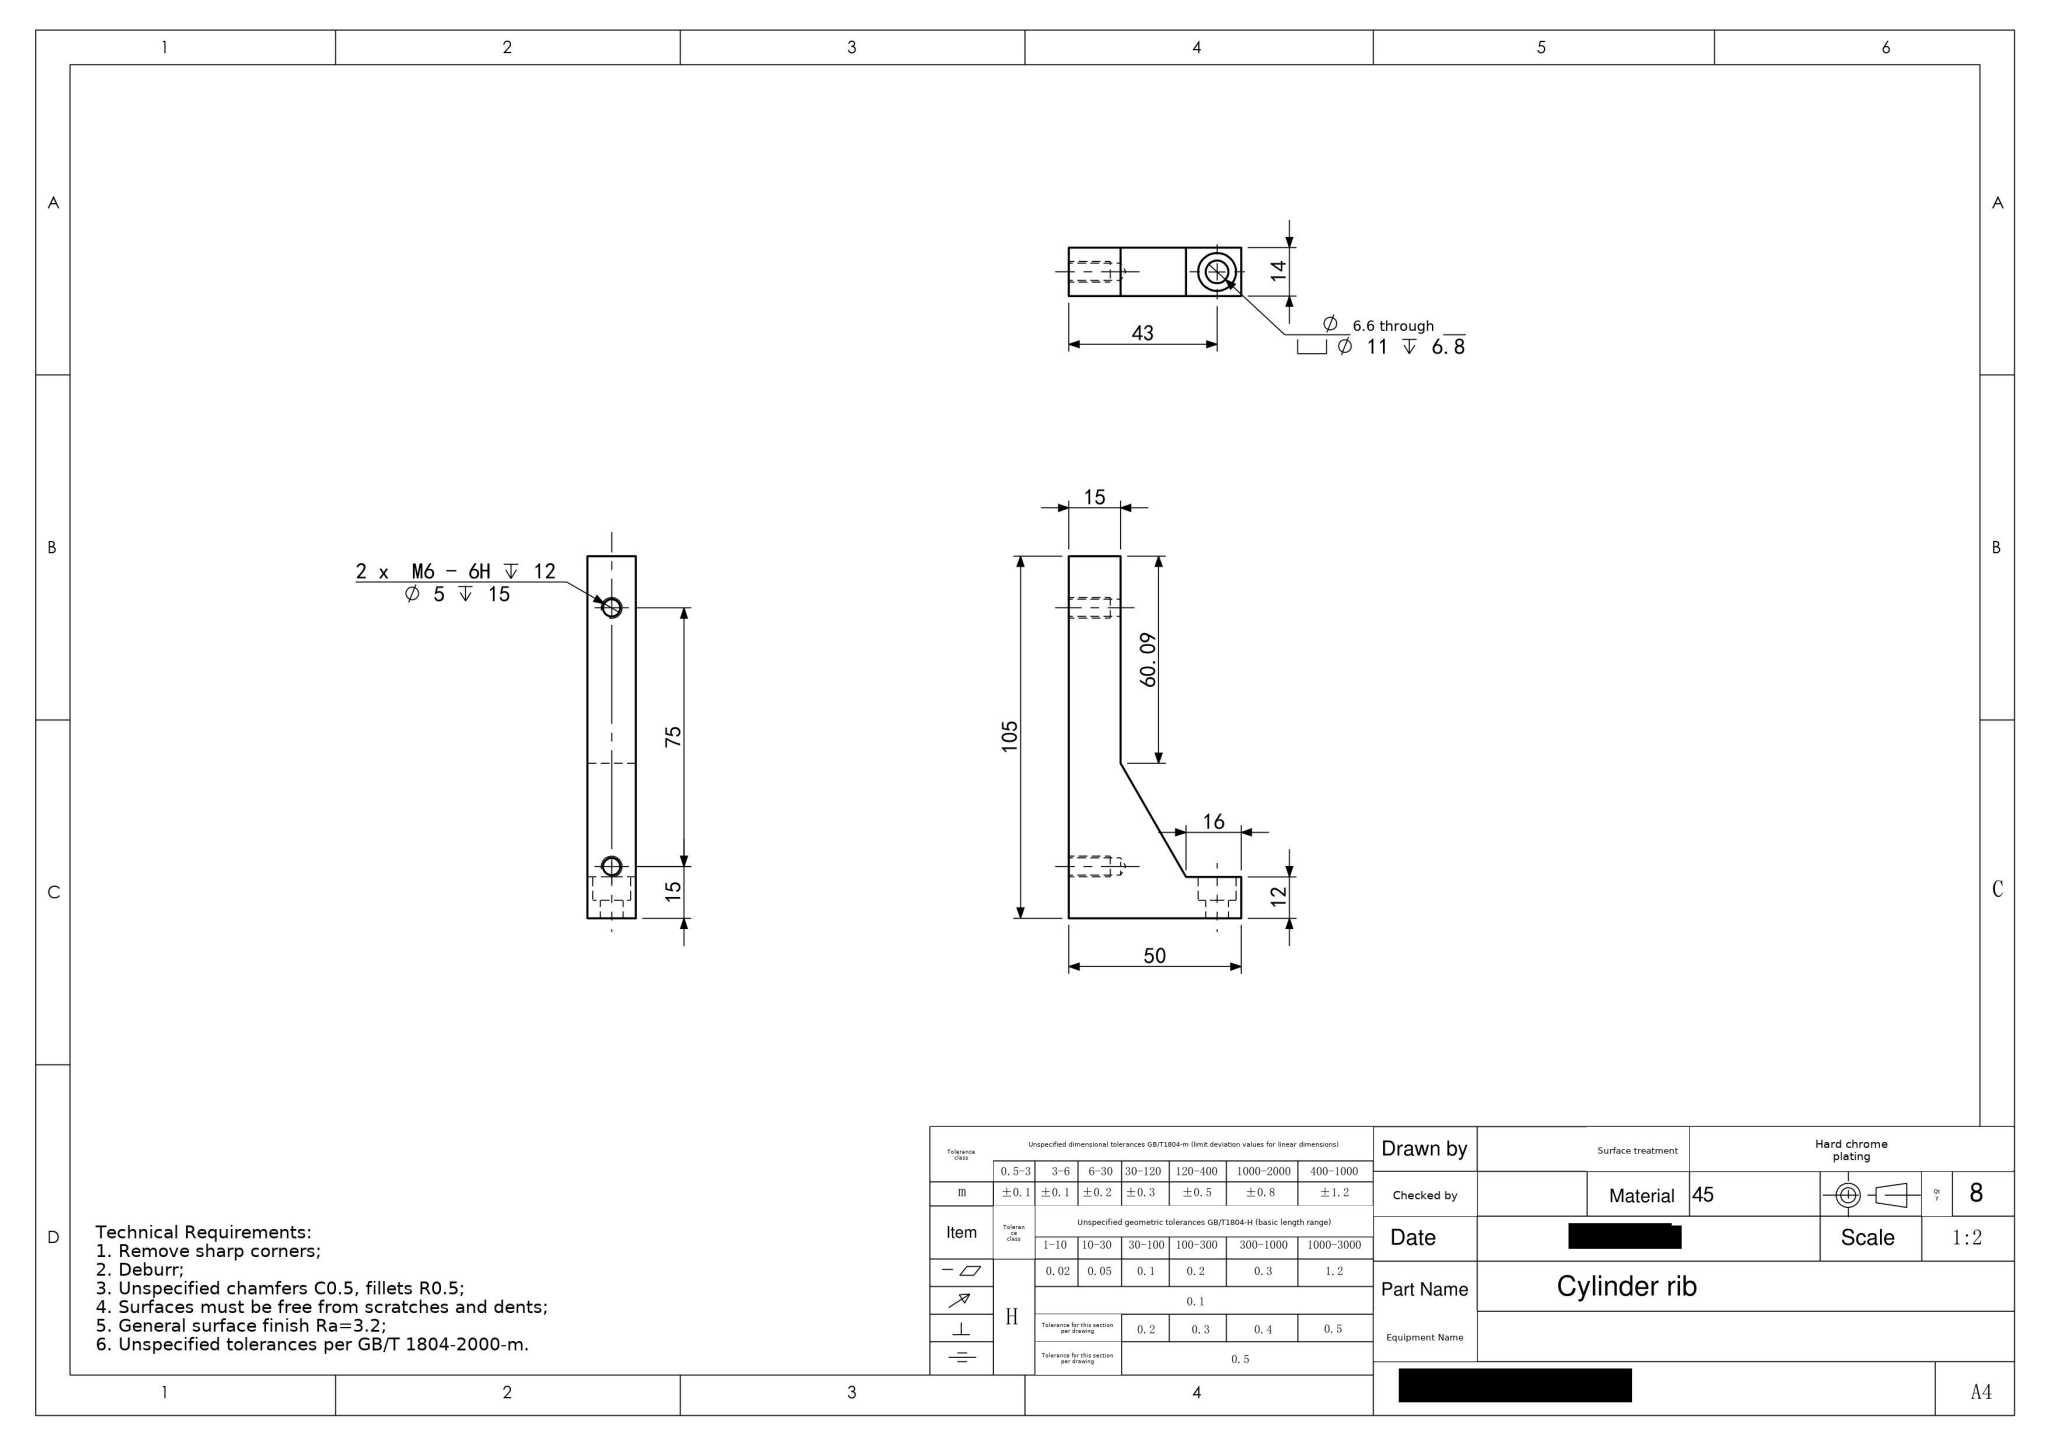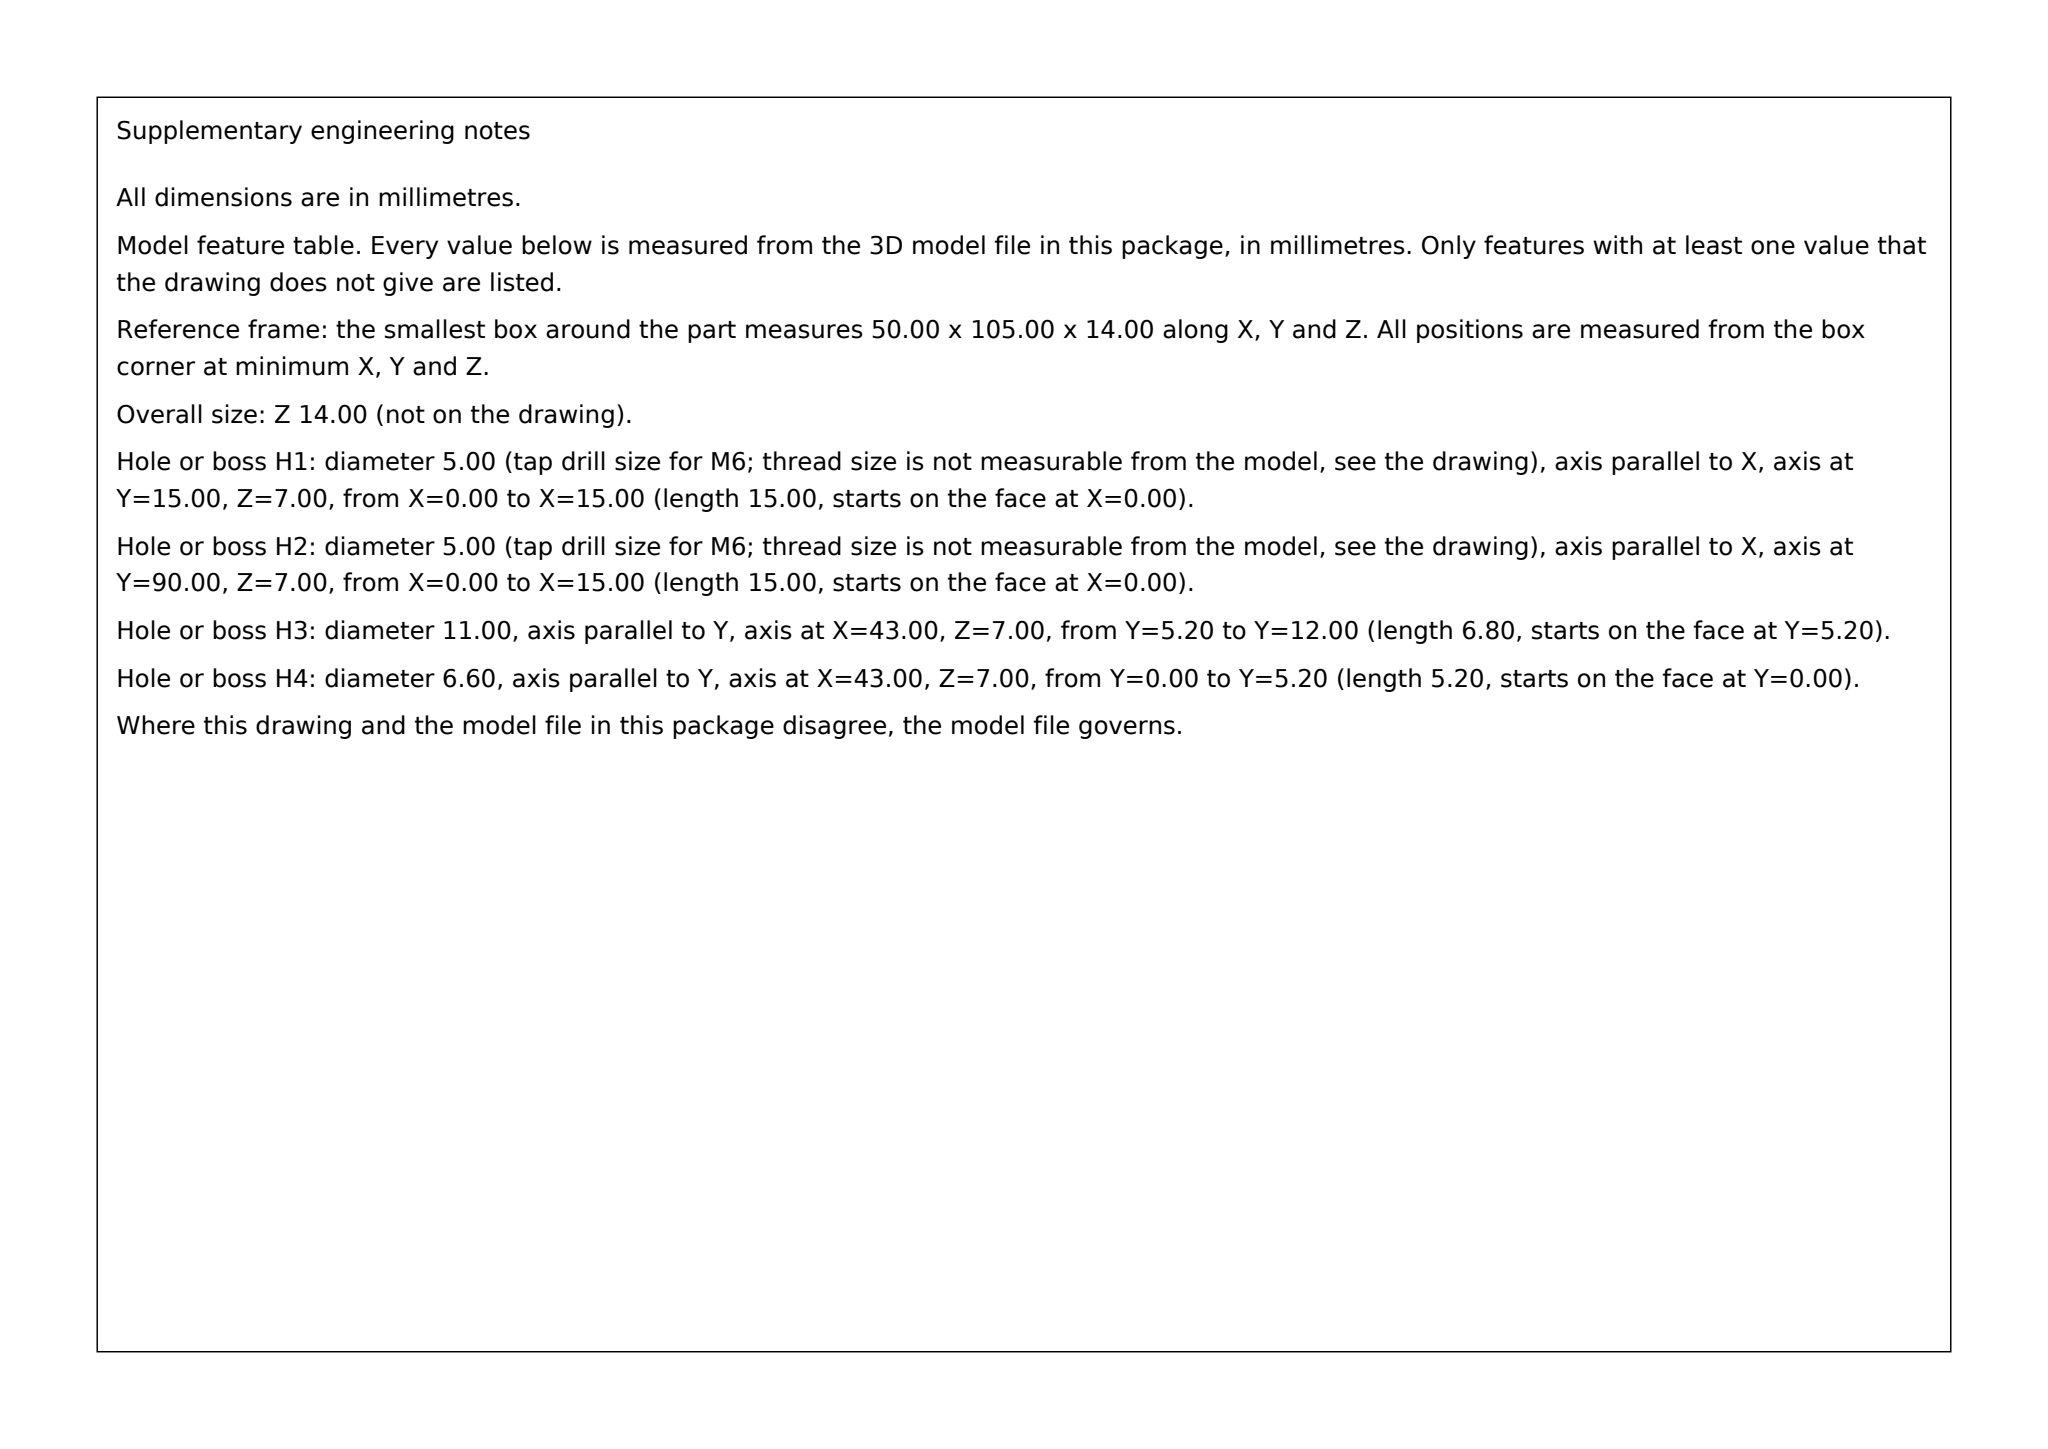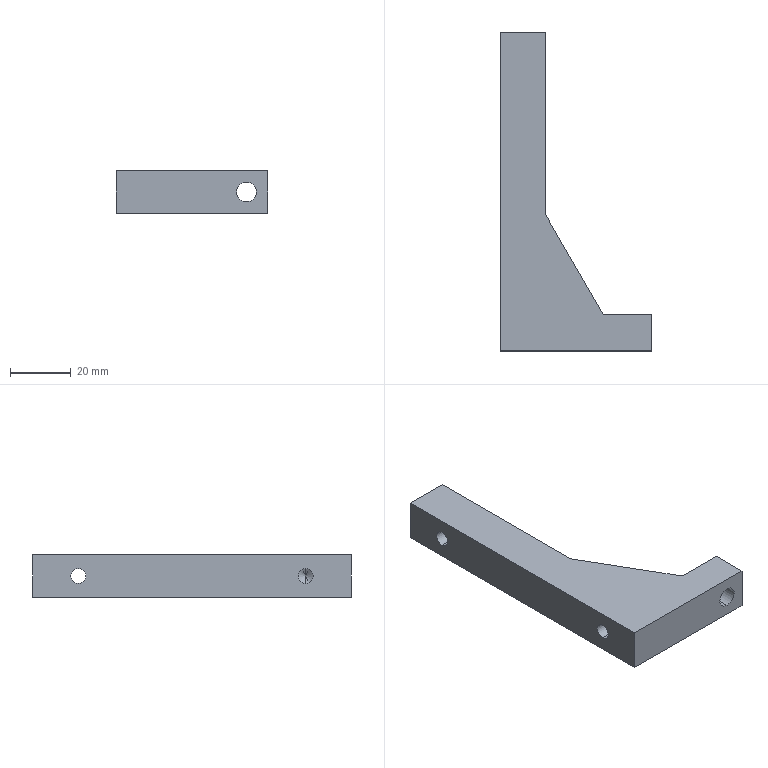Part | SolidWorks | mm | material 45 | 1 solid | 20 faces | box 50 x 105 x 14 mm | volume 30884 mm3 | plane 10 | cylinder 8 | cone 2 | commonest cylinder face diameters 5 x4 11 x2 6.6 x2
build123d program:
from build123d import *

# Parameters (mm, degrees)
BOSS_EXTRUDE1_DEPTH                             = 7
M6_HEX_SOCKET_HEAD_CAP_SCREW_CBORE1_D           = 6.6
M6_HEX_SOCKET_HEAD_CAP_SCREW_CBORE1_CBORE_D     = 11
M6_HEX_SOCKET_HEAD_CAP_SCREW_CBORE1_CBORE_DEPTH = 6.8
LPATTERN1_COUNT                                 = 2
LPATTERN1_PITCH                                 = 75


with BuildPart() as part:
    # Sketch1 → Boss-Extrude1 (new, symmetric)
    with BuildSketch(Plane.XY):
        Polygon((-25, 0), (25, 0), (25, 12), (9, 12), (-10, 44.909), (-10, 105), (-25, 105), align=None)
    extrude(amount=BOSS_EXTRUDE1_DEPTH, both=True)

    # M6 Hex Socket Head Cap Screw CBORE1 (through all)
    with Locations(Plane(origin=(0, 12, 0), x_dir=(1, 0, 0), z_dir=(0, 1, 0))):
        with Locations((18, 0)):
            CounterBoreHole(M6_HEX_SOCKET_HEAD_CAP_SCREW_CBORE1_D / 2, M6_HEX_SOCKET_HEAD_CAP_SCREW_CBORE1_CBORE_D / 2, M6_HEX_SOCKET_HEAD_CAP_SCREW_CBORE1_CBORE_DEPTH)

    # Sketch5 → M6 Tapped Hole1 (revolve, cut)
    with BuildSketch(Plane(origin=(-25, 90, 0), x_dir=(0, 0, 1), z_dir=(0, 1, 0))):
        Polygon((0, 0), (0, 16.502), (2.5, 15), (2.5, 0), align=None)
    m6_tapped_hole1 = revolve(axis=Axis((-31.35, 90, 0), (1, 0, 0)), mode=Mode.SUBTRACT)

    # LPattern1: M6 Tapped Hole1 ×2
    with Locations(*[(0, -i * LPATTERN1_PITCH, 0) for i in range(1, LPATTERN1_COUNT)]):
        add(m6_tapped_hole1, mode=Mode.SUBTRACT)


solid = part.part
STEP:
#1=CARTESIAN_POINT('',(-10.,15.,-2.5));
#2=VERTEX_POINT('',#1);
#3=CARTESIAN_POINT('',(-10.,15.,2.5));
#4=VERTEX_POINT('',#3);
#5=CARTESIAN_POINT('',(-10.,15.,0.));
#6=DIRECTION('',(-1.,0.,0.));
#7=DIRECTION('',(0.,0.,1.));
#8=AXIS2_PLACEMENT_3D('',#5,#6,#7);
#9=CIRCLE('',#8,2.5);
#10=EDGE_CURVE('',#2,#4,#9,.T.);
#11=ORIENTED_EDGE('',*,*,#10,.F.);
#12=CARTESIAN_POINT('',(-25.,15.,-2.5));
#13=VERTEX_POINT('',#12);
#14=CARTESIAN_POINT('',(-25.,15.,-2.5));
#15=DIRECTION('',(-1.,0.,0.));
#16=VECTOR('',#15,1000.);
#17=LINE('',#14,#16);
#18=EDGE_CURVE('',#2,#13,#17,.T.);
#19=ORIENTED_EDGE('',*,*,#18,.T.);
#20=CARTESIAN_POINT('',(-25.,15.,2.5));
#21=VERTEX_POINT('',#20);
#22=CARTESIAN_POINT('',(-25.,15.,0.));
#23=DIRECTION('',(-1.,0.,0.));
#24=DIRECTION('',(0.,0.,1.));
#25=AXIS2_PLACEMENT_3D('',#22,#23,#24);
#26=CIRCLE('',#25,2.5);
#27=EDGE_CURVE('',#13,#21,#26,.T.);
#28=ORIENTED_EDGE('',*,*,#27,.T.);
#29=CARTESIAN_POINT('',(-25.,15.,2.5));
#30=DIRECTION('',(-1.,0.,0.));
#31=VECTOR('',#30,1000.);
#32=LINE('',#29,#31);
#33=EDGE_CURVE('',#4,#21,#32,.T.);
#34=ORIENTED_EDGE('',*,*,#33,.F.);
#35=EDGE_LOOP('',(#11,#19,#28,#34));
#36=FACE_OUTER_BOUND('',#35,.T.);
#37=CARTESIAN_POINT('',(-25.,15.,0.));
#38=DIRECTION('',(-1.,0.,0.));
#39=DIRECTION('',(0.,0.,1.));
#40=AXIS2_PLACEMENT_3D('',#37,#38,#39);
#41=CYLINDRICAL_SURFACE('',#40,2.5);
#42=ADVANCED_FACE('',(#36),#41,.F.);
#43=CARTESIAN_POINT('',(-8.498,15.,0.));
#44=VERTEX_POINT('',#43);
#45=CARTESIAN_POINT('',(-10.,15.,2.5));
#46=DIRECTION('',(-0.515,0.,0.8572));
#47=VECTOR('',#46,1000.);
#48=LINE('',#45,#47);
#49=EDGE_CURVE('',#44,#4,#48,.T.);
#50=ORIENTED_EDGE('',*,*,#49,.F.);
#51=CARTESIAN_POINT('',(-10.,15.,-2.5));
#52=DIRECTION('',(-0.515,0.,-0.8572));
#53=VECTOR('',#52,1000.);
#54=LINE('',#51,#53);
#55=EDGE_CURVE('',#44,#2,#54,.T.);
#56=ORIENTED_EDGE('',*,*,#55,.T.);
#57=ORIENTED_EDGE('',*,*,#10,.T.);
#58=EDGE_LOOP('',(#50,#56,#57));
#59=FACE_OUTER_BOUND('',#58,.T.);
#60=CARTESIAN_POINT('',(-10.,15.,0.));
#61=DIRECTION('',(-1.,0.,0.));
#62=DIRECTION('',(0.,0.,1.));
#63=AXIS2_PLACEMENT_3D('',#60,#61,#62);
#64=CONICAL_SURFACE('',#63,2.5,1.03);
#65=ADVANCED_FACE('',(#59),#64,.F.);
#66=CARTESIAN_POINT('',(-10.,90.,-2.5));
#67=VERTEX_POINT('',#66);
#68=CARTESIAN_POINT('',(-10.,90.,2.5));
#69=VERTEX_POINT('',#68);
#70=CARTESIAN_POINT('',(-10.,90.,0.));
#71=DIRECTION('',(-1.,0.,0.));
#72=DIRECTION('',(0.,0.,1.));
#73=AXIS2_PLACEMENT_3D('',#70,#71,#72);
#74=CIRCLE('',#73,2.5);
#75=EDGE_CURVE('',#67,#69,#74,.T.);
#76=ORIENTED_EDGE('',*,*,#75,.F.);
#77=CARTESIAN_POINT('',(-25.,90.,-2.5));
#78=VERTEX_POINT('',#77);
#79=CARTESIAN_POINT('',(-25.,90.,-2.5));
#80=DIRECTION('',(-1.,0.,0.));
#81=VECTOR('',#80,1000.);
#82=LINE('',#79,#81);
#83=EDGE_CURVE('',#67,#78,#82,.T.);
#84=ORIENTED_EDGE('',*,*,#83,.T.);
#85=CARTESIAN_POINT('',(-25.,90.,2.5));
#86=VERTEX_POINT('',#85);
#87=CARTESIAN_POINT('',(-25.,90.,0.));
#88=DIRECTION('',(-1.,0.,0.));
#89=DIRECTION('',(0.,0.,1.));
#90=AXIS2_PLACEMENT_3D('',#87,#88,#89);
#91=CIRCLE('',#90,2.5);
#92=EDGE_CURVE('',#78,#86,#91,.T.);
#93=ORIENTED_EDGE('',*,*,#92,.T.);
#94=CARTESIAN_POINT('',(-25.,90.,2.5));
#95=DIRECTION('',(-1.,0.,0.));
#96=VECTOR('',#95,1000.);
#97=LINE('',#94,#96);
#98=EDGE_CURVE('',#69,#86,#97,.T.);
#99=ORIENTED_EDGE('',*,*,#98,.F.);
#100=EDGE_LOOP('',(#76,#84,#93,#99));
#101=FACE_OUTER_BOUND('',#100,.T.);
#102=CARTESIAN_POINT('',(-25.,90.,0.));
#103=DIRECTION('',(-1.,0.,0.));
#104=DIRECTION('',(0.,0.,1.));
#105=AXIS2_PLACEMENT_3D('',#102,#103,#104);
#106=CYLINDRICAL_SURFACE('',#105,2.5);
#107=ADVANCED_FACE('',(#101),#106,.F.);
#108=CARTESIAN_POINT('',(18.,5.2,-5.5));
#109=VERTEX_POINT('',#108);
#110=CARTESIAN_POINT('',(18.,5.2,5.5));
#111=VERTEX_POINT('',#110);
#112=CARTESIAN_POINT('',(18.,5.2,0.));
#113=DIRECTION('',(0.,1.,0.));
#114=DIRECTION('',(0.,0.,1.));
#115=AXIS2_PLACEMENT_3D('',#112,#113,#114);
#116=CIRCLE('',#115,5.5);
#117=EDGE_CURVE('',#109,#111,#116,.T.);
#118=ORIENTED_EDGE('',*,*,#117,.F.);
#119=CARTESIAN_POINT('',(18.,12.,-5.5));
#120=VERTEX_POINT('',#119);
#121=CARTESIAN_POINT('',(18.,12.,-5.5));
#122=DIRECTION('',(0.,1.,0.));
#123=VECTOR('',#122,1000.);
#124=LINE('',#121,#123);
#125=EDGE_CURVE('',#109,#120,#124,.T.);
#126=ORIENTED_EDGE('',*,*,#125,.T.);
#127=CARTESIAN_POINT('',(18.,12.,5.5));
#128=VERTEX_POINT('',#127);
#129=CARTESIAN_POINT('',(18.,12.,0.));
#130=DIRECTION('',(0.,1.,0.));
#131=DIRECTION('',(0.,0.,1.));
#132=AXIS2_PLACEMENT_3D('',#129,#130,#131);
#133=CIRCLE('',#132,5.5);
#134=EDGE_CURVE('',#120,#128,#133,.T.);
#135=ORIENTED_EDGE('',*,*,#134,.T.);
#136=CARTESIAN_POINT('',(18.,12.,5.5));
#137=DIRECTION('',(0.,1.,0.));
#138=VECTOR('',#137,1000.);
#139=LINE('',#136,#138);
#140=EDGE_CURVE('',#111,#128,#139,.T.);
#141=ORIENTED_EDGE('',*,*,#140,.F.);
#142=EDGE_LOOP('',(#118,#126,#135,#141));
#143=FACE_OUTER_BOUND('',#142,.T.);
#144=CARTESIAN_POINT('',(18.,12.,0.));
#145=DIRECTION('',(0.,1.,0.));
#146=DIRECTION('',(0.,0.,1.));
#147=AXIS2_PLACEMENT_3D('',#144,#145,#146);
#148=CYLINDRICAL_SURFACE('',#147,5.5);
#149=ADVANCED_FACE('',(#143),#148,.F.);
#150=CARTESIAN_POINT('',(18.,0.,-3.3));
#151=VERTEX_POINT('',#150);
#152=CARTESIAN_POINT('',(18.,0.,3.3));
#153=VERTEX_POINT('',#152);
#154=CARTESIAN_POINT('',(18.,0.,0.));
#155=DIRECTION('',(-0.,1.,0.));
#156=DIRECTION('',(-1.,-0.,0.));
#157=AXIS2_PLACEMENT_3D('',#154,#155,#156);
#158=CIRCLE('',#157,3.3);
#159=EDGE_CURVE('',#151,#153,#158,.T.);
#160=ORIENTED_EDGE('',*,*,#159,.F.);
#161=CARTESIAN_POINT('',(18.,5.2,-3.3));
#162=VERTEX_POINT('',#161);
#163=CARTESIAN_POINT('',(18.,12.,-3.3));
#164=DIRECTION('',(0.,1.,0.));
#165=VECTOR('',#164,1000.);
#166=LINE('',#163,#165);
#167=EDGE_CURVE('',#151,#162,#166,.T.);
#168=ORIENTED_EDGE('',*,*,#167,.T.);
#169=CARTESIAN_POINT('',(18.,5.2,3.3));
#170=VERTEX_POINT('',#169);
#171=CARTESIAN_POINT('',(18.,5.2,0.));
#172=DIRECTION('',(0.,1.,0.));
#173=DIRECTION('',(0.,0.,1.));
#174=AXIS2_PLACEMENT_3D('',#171,#172,#173);
#175=CIRCLE('',#174,3.3);
#176=EDGE_CURVE('',#162,#170,#175,.T.);
#177=ORIENTED_EDGE('',*,*,#176,.T.);
#178=CARTESIAN_POINT('',(18.,12.,3.3));
#179=DIRECTION('',(0.,1.,0.));
#180=VECTOR('',#179,1000.);
#181=LINE('',#178,#180);
#182=EDGE_CURVE('',#153,#170,#181,.T.);
#183=ORIENTED_EDGE('',*,*,#182,.F.);
#184=EDGE_LOOP('',(#160,#168,#177,#183));
#185=FACE_OUTER_BOUND('',#184,.T.);
#186=CARTESIAN_POINT('',(18.,12.,0.));
#187=DIRECTION('',(0.,1.,0.));
#188=DIRECTION('',(0.,0.,1.));
#189=AXIS2_PLACEMENT_3D('',#186,#187,#188);
#190=CYLINDRICAL_SURFACE('',#189,3.3);
#191=ADVANCED_FACE('',(#185),#190,.F.);
#192=CARTESIAN_POINT('',(-25.,15.,0.));
#193=DIRECTION('',(-1.,0.,0.));
#194=DIRECTION('',(0.,0.,1.));
#195=AXIS2_PLACEMENT_3D('',#192,#193,#194);
#196=CIRCLE('',#195,2.5);
#197=EDGE_CURVE('',#21,#13,#196,.T.);
#198=ORIENTED_EDGE('',*,*,#197,.F.);
#199=ORIENTED_EDGE('',*,*,#27,.F.);
#200=EDGE_LOOP('',(#198,#199));
#201=FACE_BOUND('',#200,.T.);
#202=CARTESIAN_POINT('',(-25.,90.,0.));
#203=DIRECTION('',(-1.,0.,0.));
#204=DIRECTION('',(0.,0.,1.));
#205=AXIS2_PLACEMENT_3D('',#202,#203,#204);
#206=CIRCLE('',#205,2.5);
#207=EDGE_CURVE('',#86,#78,#206,.T.);
#208=ORIENTED_EDGE('',*,*,#207,.F.);
#209=ORIENTED_EDGE('',*,*,#92,.F.);
#210=EDGE_LOOP('',(#208,#209));
#211=FACE_BOUND('',#210,.T.);
#212=CARTESIAN_POINT('',(-25.,105.,-7.));
#213=VERTEX_POINT('',#212);
#214=CARTESIAN_POINT('',(-25.,0.,-7.));
#215=VERTEX_POINT('',#214);
#216=CARTESIAN_POINT('',(-25.,0.,-7.));
#217=DIRECTION('',(0.,-1.,0.));
#218=VECTOR('',#217,1000.);
#219=LINE('',#216,#218);
#220=EDGE_CURVE('',#213,#215,#219,.T.);
#221=ORIENTED_EDGE('',*,*,#220,.T.);
#222=CARTESIAN_POINT('',(-25.,0.,7.));
#223=VERTEX_POINT('',#222);
#224=CARTESIAN_POINT('',(-25.,0.,7.));
#225=DIRECTION('',(0.,0.,-1.));
#226=VECTOR('',#225,1000.);
#227=LINE('',#224,#226);
#228=EDGE_CURVE('',#223,#215,#227,.T.);
#229=ORIENTED_EDGE('',*,*,#228,.F.);
#230=CARTESIAN_POINT('',(-25.,105.,7.));
#231=VERTEX_POINT('',#230);
#232=CARTESIAN_POINT('',(-25.,0.,7.));
#233=DIRECTION('',(0.,-1.,0.));
#234=VECTOR('',#233,1000.);
#235=LINE('',#232,#234);
#236=EDGE_CURVE('',#231,#223,#235,.T.);
#237=ORIENTED_EDGE('',*,*,#236,.F.);
#238=CARTESIAN_POINT('',(-25.,105.,7.));
#239=DIRECTION('',(0.,0.,-1.));
#240=VECTOR('',#239,1000.);
#241=LINE('',#238,#240);
#242=EDGE_CURVE('',#231,#213,#241,.T.);
#243=ORIENTED_EDGE('',*,*,#242,.T.);
#244=EDGE_LOOP('',(#221,#229,#237,#243));
#245=FACE_OUTER_BOUND('',#244,.T.);
#246=CARTESIAN_POINT('',(-25.,0.,7.));
#247=DIRECTION('',(1.,0.,0.));
#248=DIRECTION('',(0.,0.,-1.));
#249=AXIS2_PLACEMENT_3D('',#246,#247,#248);
#250=PLANE('',#249);
#251=ADVANCED_FACE('',(#201,#211,#245),#250,.F.);
#252=CARTESIAN_POINT('',(18.,0.,0.));
#253=DIRECTION('',(-0.,1.,0.));
#254=DIRECTION('',(-1.,-0.,0.));
#255=AXIS2_PLACEMENT_3D('',#252,#253,#254);
#256=CIRCLE('',#255,3.3);
#257=EDGE_CURVE('',#153,#151,#256,.T.);
#258=ORIENTED_EDGE('',*,*,#257,.T.);
#259=ORIENTED_EDGE('',*,*,#159,.T.);
#260=EDGE_LOOP('',(#258,#259));
#261=FACE_BOUND('',#260,.T.);
#262=CARTESIAN_POINT('',(25.,0.,-7.));
#263=VERTEX_POINT('',#262);
#264=CARTESIAN_POINT('',(-25.,0.,-7.));
#265=DIRECTION('',(1.,0.,0.));
#266=VECTOR('',#265,1000.);
#267=LINE('',#264,#266);
#268=EDGE_CURVE('',#215,#263,#267,.T.);
#269=ORIENTED_EDGE('',*,*,#268,.T.);
#270=CARTESIAN_POINT('',(25.,0.,7.));
#271=VERTEX_POINT('',#270);
#272=CARTESIAN_POINT('',(25.,0.,7.));
#273=DIRECTION('',(0.,0.,-1.));
#274=VECTOR('',#273,1000.);
#275=LINE('',#272,#274);
#276=EDGE_CURVE('',#271,#263,#275,.T.);
#277=ORIENTED_EDGE('',*,*,#276,.F.);
#278=CARTESIAN_POINT('',(-25.,0.,7.));
#279=DIRECTION('',(1.,0.,0.));
#280=VECTOR('',#279,1000.);
#281=LINE('',#278,#280);
#282=EDGE_CURVE('',#223,#271,#281,.T.);
#283=ORIENTED_EDGE('',*,*,#282,.F.);
#284=ORIENTED_EDGE('',*,*,#228,.T.);
#285=EDGE_LOOP('',(#269,#277,#283,#284));
#286=FACE_OUTER_BOUND('',#285,.T.);
#287=CARTESIAN_POINT('',(-25.,0.,7.));
#288=DIRECTION('',(-0.,1.,0.));
#289=DIRECTION('',(-1.,-0.,0.));
#290=AXIS2_PLACEMENT_3D('',#287,#288,#289);
#291=PLANE('',#290);
#292=ADVANCED_FACE('',(#261,#286),#291,.F.);
#293=CARTESIAN_POINT('',(25.,12.,-7.));
#294=VERTEX_POINT('',#293);
#295=CARTESIAN_POINT('',(25.,0.,-7.));
#296=DIRECTION('',(0.,1.,0.));
#297=VECTOR('',#296,1000.);
#298=LINE('',#295,#297);
#299=EDGE_CURVE('',#263,#294,#298,.T.);
#300=ORIENTED_EDGE('',*,*,#299,.T.);
#301=CARTESIAN_POINT('',(25.,12.,7.));
#302=VERTEX_POINT('',#301);
#303=CARTESIAN_POINT('',(25.,12.,7.));
#304=DIRECTION('',(0.,0.,-1.));
#305=VECTOR('',#304,1000.);
#306=LINE('',#303,#305);
#307=EDGE_CURVE('',#302,#294,#306,.T.);
#308=ORIENTED_EDGE('',*,*,#307,.F.);
#309=CARTESIAN_POINT('',(25.,0.,7.));
#310=DIRECTION('',(0.,1.,0.));
#311=VECTOR('',#310,1000.);
#312=LINE('',#309,#311);
#313=EDGE_CURVE('',#271,#302,#312,.T.);
#314=ORIENTED_EDGE('',*,*,#313,.F.);
#315=ORIENTED_EDGE('',*,*,#276,.T.);
#316=EDGE_LOOP('',(#300,#308,#314,#315));
#317=FACE_OUTER_BOUND('',#316,.T.);
#318=CARTESIAN_POINT('',(25.,0.,7.));
#319=DIRECTION('',(-1.,0.,0.));
#320=DIRECTION('',(-0.,-1.,0.));
#321=AXIS2_PLACEMENT_3D('',#318,#319,#320);
#322=PLANE('',#321);
#323=ADVANCED_FACE('',(#317),#322,.F.);
#324=CARTESIAN_POINT('',(18.,12.,0.));
#325=DIRECTION('',(0.,1.,0.));
#326=DIRECTION('',(0.,0.,1.));
#327=AXIS2_PLACEMENT_3D('',#324,#325,#326);
#328=CIRCLE('',#327,5.5);
#329=EDGE_CURVE('',#128,#120,#328,.T.);
#330=ORIENTED_EDGE('',*,*,#329,.F.);
#331=ORIENTED_EDGE('',*,*,#134,.F.);
#332=EDGE_LOOP('',(#330,#331));
#333=FACE_BOUND('',#332,.T.);
#334=CARTESIAN_POINT('',(9.,12.,-7.));
#335=VERTEX_POINT('',#334);
#336=CARTESIAN_POINT('',(9.,12.,-7.));
#337=DIRECTION('',(-1.,0.,0.));
#338=VECTOR('',#337,1000.);
#339=LINE('',#336,#338);
#340=EDGE_CURVE('',#294,#335,#339,.T.);
#341=ORIENTED_EDGE('',*,*,#340,.T.);
#342=CARTESIAN_POINT('',(9.,12.,7.));
#343=VERTEX_POINT('',#342);
#344=CARTESIAN_POINT('',(9.,12.,7.));
#345=DIRECTION('',(0.,0.,-1.));
#346=VECTOR('',#345,1000.);
#347=LINE('',#344,#346);
#348=EDGE_CURVE('',#343,#335,#347,.T.);
#349=ORIENTED_EDGE('',*,*,#348,.F.);
#350=CARTESIAN_POINT('',(9.,12.,7.));
#351=DIRECTION('',(-1.,0.,0.));
#352=VECTOR('',#351,1000.);
#353=LINE('',#350,#352);
#354=EDGE_CURVE('',#302,#343,#353,.T.);
#355=ORIENTED_EDGE('',*,*,#354,.F.);
#356=ORIENTED_EDGE('',*,*,#307,.T.);
#357=EDGE_LOOP('',(#341,#349,#355,#356));
#358=FACE_OUTER_BOUND('',#357,.T.);
#359=CARTESIAN_POINT('',(9.,12.,7.));
#360=DIRECTION('',(0.,-1.,0.));
#361=DIRECTION('',(0.,0.,-1.));
#362=AXIS2_PLACEMENT_3D('',#359,#360,#361);
#363=PLANE('',#362);
#364=ADVANCED_FACE('',(#333,#358),#363,.F.);
#365=CARTESIAN_POINT('',(-10.,44.909,-7.));
#366=VERTEX_POINT('',#365);
#367=CARTESIAN_POINT('',(-10.,44.909,-7.));
#368=DIRECTION('',(-0.5,0.866,0.));
#369=VECTOR('',#368,1000.);
#370=LINE('',#367,#369);
#371=EDGE_CURVE('',#335,#366,#370,.T.);
#372=ORIENTED_EDGE('',*,*,#371,.T.);
#373=CARTESIAN_POINT('',(-10.,44.909,7.));
#374=VERTEX_POINT('',#373);
#375=CARTESIAN_POINT('',(-10.,44.909,7.));
#376=DIRECTION('',(0.,0.,-1.));
#377=VECTOR('',#376,1000.);
#378=LINE('',#375,#377);
#379=EDGE_CURVE('',#374,#366,#378,.T.);
#380=ORIENTED_EDGE('',*,*,#379,.F.);
#381=CARTESIAN_POINT('',(-10.,44.909,7.));
#382=DIRECTION('',(-0.5,0.866,0.));
#383=VECTOR('',#382,1000.);
#384=LINE('',#381,#383);
#385=EDGE_CURVE('',#343,#374,#384,.T.);
#386=ORIENTED_EDGE('',*,*,#385,.F.);
#387=ORIENTED_EDGE('',*,*,#348,.T.);
#388=EDGE_LOOP('',(#372,#380,#386,#387));
#389=FACE_OUTER_BOUND('',#388,.T.);
#390=CARTESIAN_POINT('',(-10.,44.909,7.));
#391=DIRECTION('',(-0.866,-0.5,0.));
#392=DIRECTION('',(0.5,-0.866,0.));
#393=AXIS2_PLACEMENT_3D('',#390,#391,#392);
#394=PLANE('',#393);
#395=ADVANCED_FACE('',(#389),#394,.F.);
#396=CARTESIAN_POINT('',(-10.,90.,0.));
#397=DIRECTION('',(-1.,0.,0.));
#398=DIRECTION('',(0.,0.,1.));
#399=AXIS2_PLACEMENT_3D('',#396,#397,#398);
#400=CIRCLE('',#399,2.5);
#401=EDGE_CURVE('',#69,#67,#400,.T.);
#402=ORIENTED_EDGE('',*,*,#401,.T.);
#403=ORIENTED_EDGE('',*,*,#75,.T.);
#404=EDGE_LOOP('',(#402,#403));
#405=FACE_BOUND('',#404,.T.);
#406=CARTESIAN_POINT('',(-10.,105.,-7.));
#407=VERTEX_POINT('',#406);
#408=CARTESIAN_POINT('',(-10.,105.,-7.));
#409=DIRECTION('',(-0.,1.,0.));
#410=VECTOR('',#409,1000.);
#411=LINE('',#408,#410);
#412=EDGE_CURVE('',#366,#407,#411,.T.);
#413=ORIENTED_EDGE('',*,*,#412,.T.);
#414=CARTESIAN_POINT('',(-10.,105.,7.));
#415=VERTEX_POINT('',#414);
#416=CARTESIAN_POINT('',(-10.,105.,7.));
#417=DIRECTION('',(0.,0.,-1.));
#418=VECTOR('',#417,1000.);
#419=LINE('',#416,#418);
#420=EDGE_CURVE('',#415,#407,#419,.T.);
#421=ORIENTED_EDGE('',*,*,#420,.F.);
#422=CARTESIAN_POINT('',(-10.,105.,7.));
#423=DIRECTION('',(-0.,1.,0.));
#424=VECTOR('',#423,1000.);
#425=LINE('',#422,#424);
#426=EDGE_CURVE('',#374,#415,#425,.T.);
#427=ORIENTED_EDGE('',*,*,#426,.F.);
#428=ORIENTED_EDGE('',*,*,#379,.T.);
#429=EDGE_LOOP('',(#413,#421,#427,#428));
#430=FACE_OUTER_BOUND('',#429,.T.);
#431=CARTESIAN_POINT('',(-10.,105.,7.));
#432=DIRECTION('',(-1.,-0.,0.));
#433=DIRECTION('',(0.,-1.,0.));
#434=AXIS2_PLACEMENT_3D('',#431,#432,#433);
#435=PLANE('',#434);
#436=ADVANCED_FACE('',(#405,#430),#435,.F.);
#437=CARTESIAN_POINT('',(-25.,105.,-7.));
#438=DIRECTION('',(-1.,0.,0.));
#439=VECTOR('',#438,1000.);
#440=LINE('',#437,#439);
#441=EDGE_CURVE('',#407,#213,#440,.T.);
#442=ORIENTED_EDGE('',*,*,#441,.T.);
#443=ORIENTED_EDGE('',*,*,#242,.F.);
#444=CARTESIAN_POINT('',(-25.,105.,7.));
#445=DIRECTION('',(-1.,0.,0.));
#446=VECTOR('',#445,1000.);
#447=LINE('',#444,#446);
#448=EDGE_CURVE('',#415,#231,#447,.T.);
#449=ORIENTED_EDGE('',*,*,#448,.F.);
#450=ORIENTED_EDGE('',*,*,#420,.T.);
#451=EDGE_LOOP('',(#442,#443,#449,#450));
#452=FACE_OUTER_BOUND('',#451,.T.);
#453=CARTESIAN_POINT('',(-25.,105.,7.));
#454=DIRECTION('',(0.,-1.,0.));
#455=DIRECTION('',(0.,0.,-1.));
#456=AXIS2_PLACEMENT_3D('',#453,#454,#455);
#457=PLANE('',#456);
#458=ADVANCED_FACE('',(#452),#457,.F.);
#459=ORIENTED_EDGE('',*,*,#236,.T.);
#460=ORIENTED_EDGE('',*,*,#282,.T.);
#461=ORIENTED_EDGE('',*,*,#313,.T.);
#462=ORIENTED_EDGE('',*,*,#354,.T.);
#463=ORIENTED_EDGE('',*,*,#385,.T.);
#464=ORIENTED_EDGE('',*,*,#426,.T.);
#465=ORIENTED_EDGE('',*,*,#448,.T.);
#466=EDGE_LOOP('',(#459,#460,#461,#462,#463,#464,#465));
#467=FACE_OUTER_BOUND('',#466,.T.);
#468=CARTESIAN_POINT('',(0.,0.,7.));
#469=DIRECTION('',(0.,0.,-1.));
#470=DIRECTION('',(-1.,0.,0.));
#471=AXIS2_PLACEMENT_3D('',#468,#469,#470);
#472=PLANE('',#471);
#473=ADVANCED_FACE('',(#467),#472,.F.);
#474=ORIENTED_EDGE('',*,*,#220,.F.);
#475=ORIENTED_EDGE('',*,*,#441,.F.);
#476=ORIENTED_EDGE('',*,*,#412,.F.);
#477=ORIENTED_EDGE('',*,*,#371,.F.);
#478=ORIENTED_EDGE('',*,*,#340,.F.);
#479=ORIENTED_EDGE('',*,*,#299,.F.);
#480=ORIENTED_EDGE('',*,*,#268,.F.);
#481=EDGE_LOOP('',(#474,#475,#476,#477,#478,#479,#480));
#482=FACE_OUTER_BOUND('',#481,.T.);
#483=CARTESIAN_POINT('',(0.,0.,-7.));
#484=DIRECTION('',(0.,0.,-1.));
#485=DIRECTION('',(-1.,0.,0.));
#486=AXIS2_PLACEMENT_3D('',#483,#484,#485);
#487=PLANE('',#486);
#488=ADVANCED_FACE('',(#482),#487,.T.);
#489=ORIENTED_EDGE('',*,*,#167,.F.);
#490=ORIENTED_EDGE('',*,*,#257,.F.);
#491=ORIENTED_EDGE('',*,*,#182,.T.);
#492=CARTESIAN_POINT('',(18.,5.2,0.));
#493=DIRECTION('',(0.,1.,0.));
#494=DIRECTION('',(0.,0.,1.));
#495=AXIS2_PLACEMENT_3D('',#492,#493,#494);
#496=CIRCLE('',#495,3.3);
#497=EDGE_CURVE('',#170,#162,#496,.T.);
#498=ORIENTED_EDGE('',*,*,#497,.T.);
#499=EDGE_LOOP('',(#489,#490,#491,#498));
#500=FACE_OUTER_BOUND('',#499,.T.);
#501=CARTESIAN_POINT('',(18.,12.,0.));
#502=DIRECTION('',(0.,1.,0.));
#503=DIRECTION('',(0.,0.,1.));
#504=AXIS2_PLACEMENT_3D('',#501,#502,#503);
#505=CYLINDRICAL_SURFACE('',#504,3.3);
#506=ADVANCED_FACE('',(#500),#505,.F.);
#507=ORIENTED_EDGE('',*,*,#497,.F.);
#508=ORIENTED_EDGE('',*,*,#176,.F.);
#509=EDGE_LOOP('',(#507,#508));
#510=FACE_BOUND('',#509,.T.);
#511=CARTESIAN_POINT('',(18.,5.2,0.));
#512=DIRECTION('',(0.,1.,0.));
#513=DIRECTION('',(0.,0.,1.));
#514=AXIS2_PLACEMENT_3D('',#511,#512,#513);
#515=CIRCLE('',#514,5.5);
#516=EDGE_CURVE('',#111,#109,#515,.T.);
#517=ORIENTED_EDGE('',*,*,#516,.T.);
#518=ORIENTED_EDGE('',*,*,#117,.T.);
#519=EDGE_LOOP('',(#517,#518));
#520=FACE_OUTER_BOUND('',#519,.T.);
#521=CARTESIAN_POINT('',(21.3,5.2,0.));
#522=DIRECTION('',(0.,-1.,0.));
#523=DIRECTION('',(0.,0.,-1.));
#524=AXIS2_PLACEMENT_3D('',#521,#522,#523);
#525=PLANE('',#524);
#526=ADVANCED_FACE('',(#510,#520),#525,.F.);
#527=ORIENTED_EDGE('',*,*,#125,.F.);
#528=ORIENTED_EDGE('',*,*,#516,.F.);
#529=ORIENTED_EDGE('',*,*,#140,.T.);
#530=ORIENTED_EDGE('',*,*,#329,.T.);
#531=EDGE_LOOP('',(#527,#528,#529,#530));
#532=FACE_OUTER_BOUND('',#531,.T.);
#533=CARTESIAN_POINT('',(18.,12.,0.));
#534=DIRECTION('',(0.,1.,0.));
#535=DIRECTION('',(0.,0.,1.));
#536=AXIS2_PLACEMENT_3D('',#533,#534,#535);
#537=CYLINDRICAL_SURFACE('',#536,5.5);
#538=ADVANCED_FACE('',(#532),#537,.F.);
#539=ORIENTED_EDGE('',*,*,#83,.F.);
#540=ORIENTED_EDGE('',*,*,#401,.F.);
#541=ORIENTED_EDGE('',*,*,#98,.T.);
#542=ORIENTED_EDGE('',*,*,#207,.T.);
#543=EDGE_LOOP('',(#539,#540,#541,#542));
#544=FACE_OUTER_BOUND('',#543,.T.);
#545=CARTESIAN_POINT('',(-25.,90.,0.));
#546=DIRECTION('',(-1.,0.,0.));
#547=DIRECTION('',(0.,0.,1.));
#548=AXIS2_PLACEMENT_3D('',#545,#546,#547);
#549=CYLINDRICAL_SURFACE('',#548,2.5);
#550=ADVANCED_FACE('',(#544),#549,.F.);
#551=ORIENTED_EDGE('',*,*,#55,.F.);
#552=ORIENTED_EDGE('',*,*,#49,.T.);
#553=CARTESIAN_POINT('',(-10.,15.,0.));
#554=DIRECTION('',(-1.,0.,0.));
#555=DIRECTION('',(0.,0.,1.));
#556=AXIS2_PLACEMENT_3D('',#553,#554,#555);
#557=CIRCLE('',#556,2.5);
#558=EDGE_CURVE('',#4,#2,#557,.T.);
#559=ORIENTED_EDGE('',*,*,#558,.T.);
#560=EDGE_LOOP('',(#551,#552,#559));
#561=FACE_OUTER_BOUND('',#560,.T.);
#562=CARTESIAN_POINT('',(-10.,15.,0.));
#563=DIRECTION('',(-1.,0.,0.));
#564=DIRECTION('',(0.,0.,1.));
#565=AXIS2_PLACEMENT_3D('',#562,#563,#564);
#566=CONICAL_SURFACE('',#565,2.5,1.03);
#567=ADVANCED_FACE('',(#561),#566,.F.);
#568=ORIENTED_EDGE('',*,*,#18,.F.);
#569=ORIENTED_EDGE('',*,*,#558,.F.);
#570=ORIENTED_EDGE('',*,*,#33,.T.);
#571=ORIENTED_EDGE('',*,*,#197,.T.);
#572=EDGE_LOOP('',(#568,#569,#570,#571));
#573=FACE_OUTER_BOUND('',#572,.T.);
#574=CARTESIAN_POINT('',(-25.,15.,0.));
#575=DIRECTION('',(-1.,0.,0.));
#576=DIRECTION('',(0.,0.,1.));
#577=AXIS2_PLACEMENT_3D('',#574,#575,#576);
#578=CYLINDRICAL_SURFACE('',#577,2.5);
#579=ADVANCED_FACE('',(#573),#578,.F.);
#580=CLOSED_SHELL('',(#42,#65,#107,#149,#191,#251,#292,#323,#364,#395,#436,#458,#473,#488,#506,#526,#538,#550,#567,#579));
#581=MANIFOLD_SOLID_BREP('',#580);
#582=CARTESIAN_POINT('',(0.,0.,0.));
#583=DIRECTION('',(0.,0.,1.));
#584=DIRECTION('',(1.,0.,0.));
#585=AXIS2_PLACEMENT_3D('',#582,#583,#584);
#586=(LENGTH_UNIT()NAMED_UNIT(*)SI_UNIT(.MILLI.,.METRE.));
#587=UNCERTAINTY_MEASURE_WITH_UNIT(LENGTH_MEASURE(0.00001),#586,'','');
#588=(NAMED_UNIT(*)PLANE_ANGLE_UNIT()SI_UNIT($,.RADIAN.));
#589=(NAMED_UNIT(*)SI_UNIT($,.STERADIAN.)SOLID_ANGLE_UNIT());
#590=(GEOMETRIC_REPRESENTATION_CONTEXT(3)GLOBAL_UNCERTAINTY_ASSIGNED_CONTEXT((#587))GLOBAL_UNIT_ASSIGNED_CONTEXT((#586,#588,#589))REPRESENTATION_CONTEXT('',''));
#591=ADVANCED_BREP_SHAPE_REPRESENTATION('',(#581,#585),#590);